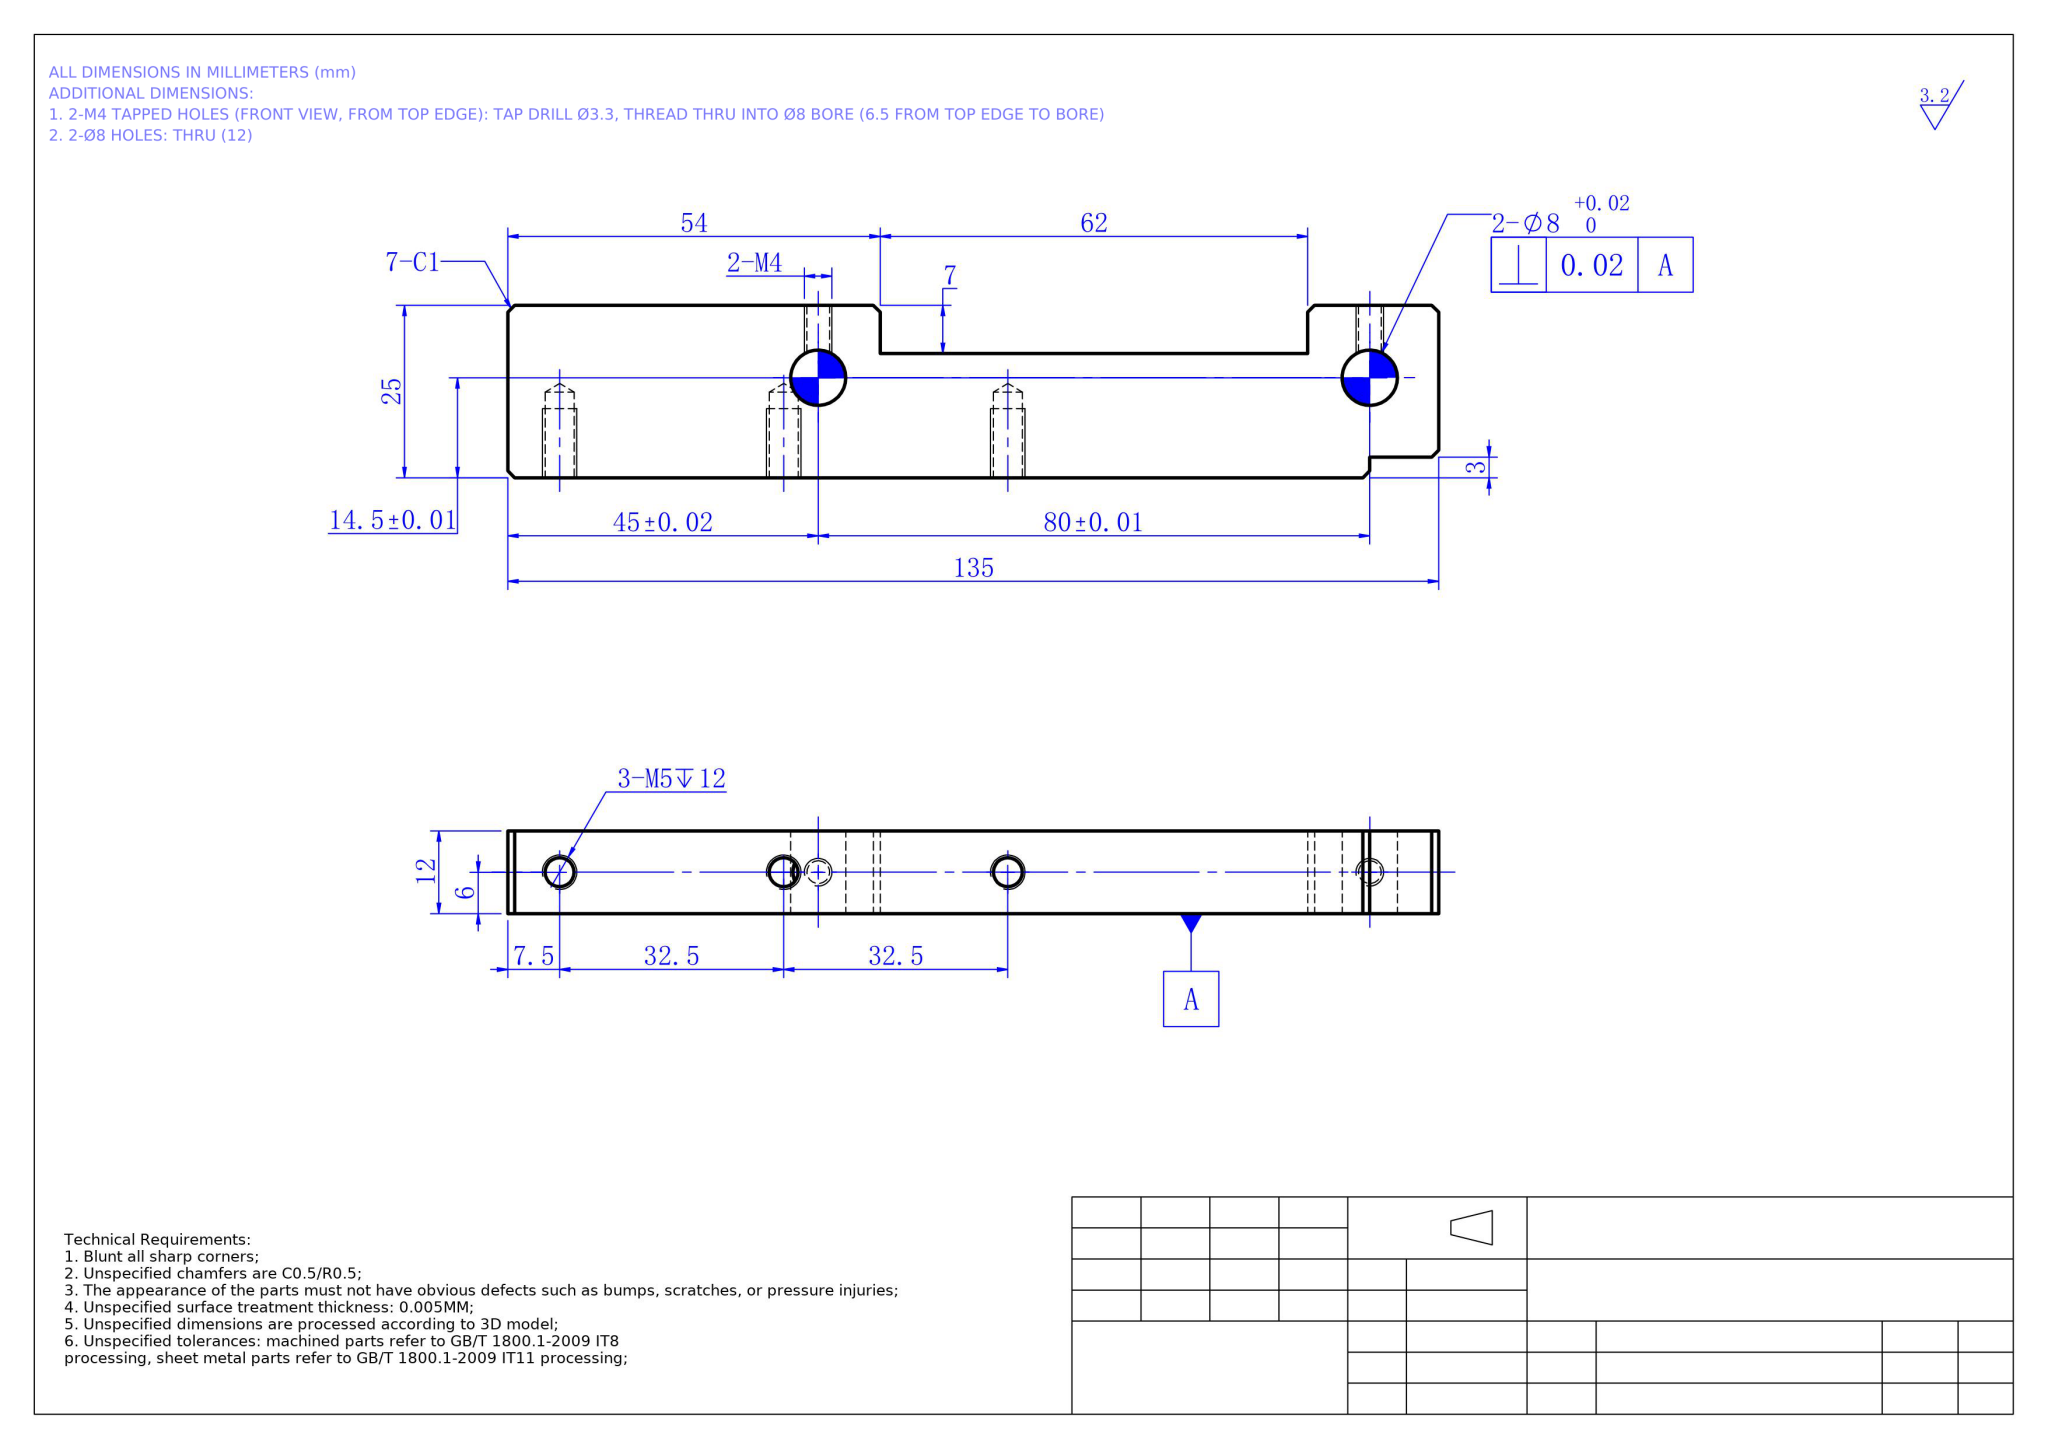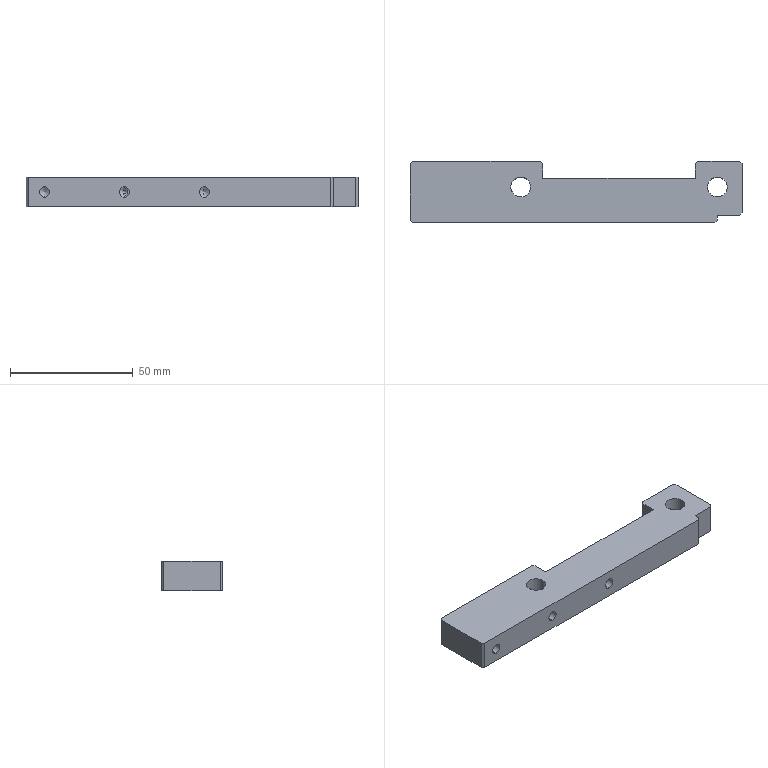Part | NX | mm | 1 solid | 39 faces | box 135 x 25 x 12 mm | volume 33039 mm3 | plane 19 | cylinder 14 | cone 6 | commonest cylinder face diameters 4.2 x6 3.3 x4 8 x4